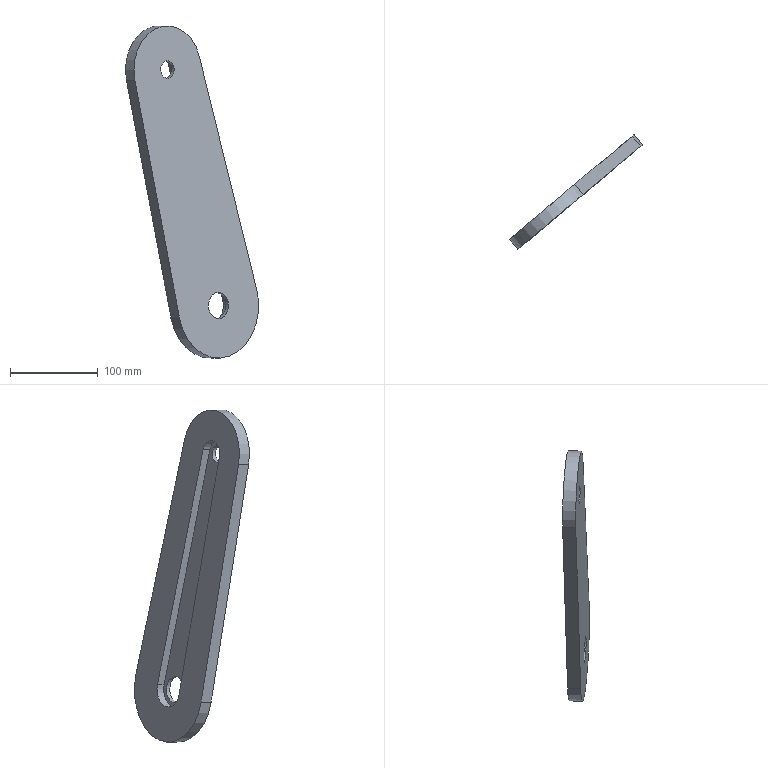Component | NX | M1002_AGO13_P09_757058_P02 | 1 solid | 13 faces | box 152.06 x 131.45 x 379.43 mm | volume 493084 mm3 | plane 7 | cylinder 6 | commonest cylinder face diameters 30 x2 20 x1 120 x1 100 x1 40 x1
STEP:
#1=CARTESIAN_POINT('',(0.,0.,0.));
#2=DIRECTION('',(0.,0.,1.));
#3=DIRECTION('',(1.,0.,0.));
#4=AXIS2_PLACEMENT_3D('',#1,#2,#3);
#5=CARTESIAN_POINT('',(13.794,-9.16,27.918));
#6=VERTEX_POINT('',#5);
#7=CARTESIAN_POINT('',(24.832,0.1404,32.));
#8=DIRECTION('',(-0.6443,0.7647,0.));
#9=DIRECTION('',(-0.7359,-0.62,-0.2721));
#10=AXIS2_PLACEMENT_3D('',#7,#8,#9);
#11=CIRCLE('',#10,15.);
#12=CARTESIAN_POINT('',(15.167,11.611,32.));
#13=DIRECTION('',(0.6443,-0.7647,0.));
#14=DIRECTION('',(-0.2081,-0.1753,0.9623));
#15=AXIS2_PLACEMENT_3D('',#12,#13,#14);
#16=CYLINDRICAL_SURFACE('',#15,15.);
#17=CARTESIAN_POINT('',(7.854,15.));
#18=DIRECTION('',(-1.,0.));
#19=VECTOR('',#18,1.);
#20=LINE('',#17,#19);
#21=(GEOMETRIC_REPRESENTATION_CONTEXT(2)PARAMETRIC_REPRESENTATION_CONTEXT()REPRESENTATION_CONTEXT('',''));
#22=DEFINITIONAL_REPRESENTATION('',(#20),#21);
#23=PCURVE('',#16,#22);
#24=CARTESIAN_POINT('',(24.832,0.1404,32.));
#25=DIRECTION('',(-0.6443,0.7647,0.));
#26=DIRECTION('',(0.2081,0.1753,-0.9623));
#27=AXIS2_PLACEMENT_3D('',#24,#25,#26);
#28=PLANE('',#27);
#29=CARTESIAN_POINT('',(0.,0.));
#30=DIRECTION('',(-0.,1.));
#31=AXIS2_PLACEMENT_2D('',#29,#30);
#32=CIRCLE('',#31,15.);
#33=(GEOMETRIC_REPRESENTATION_CONTEXT(2)PARAMETRIC_REPRESENTATION_CONTEXT()REPRESENTATION_CONTEXT('',''));
#34=DEFINITIONAL_REPRESENTATION('',(#32),#33);
#35=PCURVE('',#28,#34);
#36=SURFACE_CURVE('',#11,(#23,#35),.PCURVE_S1.);
#37=EDGE_CURVE('',#6,#6,#36,.T.);
#38=ORIENTED_EDGE('',*,*,#37,.T.);
#39=CARTESIAN_POINT('',(10.572,-5.336,27.918));
#40=VERTEX_POINT('',#39);
#41=CARTESIAN_POINT('',(10.572,-5.336,27.918));
#42=CARTESIAN_POINT('',(13.794,-9.16,27.918));
#43=B_SPLINE_CURVE_WITH_KNOTS('',1,(#41,#42),.UNSPECIFIED.,.F.,.F.,(2,2),(10.,15.),.PIECEWISE_BEZIER_KNOTS.);
#44=CARTESIAN_POINT('',(1.571,0.));
#45=DIRECTION('',(0.,1.));
#46=VECTOR('',#45,1.);
#47=LINE('',#44,#46);
#48=(GEOMETRIC_REPRESENTATION_CONTEXT(2)PARAMETRIC_REPRESENTATION_CONTEXT()REPRESENTATION_CONTEXT('',''));
#49=DEFINITIONAL_REPRESENTATION('',(#47),#48);
#50=PCURVE('',#16,#49);
#51=CARTESIAN_POINT('',(7.854,0.));
#52=DIRECTION('',(0.,1.));
#53=VECTOR('',#52,1.);
#54=LINE('',#51,#53);
#55=(GEOMETRIC_REPRESENTATION_CONTEXT(2)PARAMETRIC_REPRESENTATION_CONTEXT()REPRESENTATION_CONTEXT('',''));
#56=DEFINITIONAL_REPRESENTATION('',(#54),#55);
#57=PCURVE('',#16,#56);
#58=SEAM_CURVE('',#43,(#50,#57),.PCURVE_S1.);
#59=EDGE_CURVE('',#40,#6,#58,.T.);
#60=ORIENTED_EDGE('',*,*,#59,.F.);
#61=CARTESIAN_POINT('',(21.61,3.964,32.));
#62=DIRECTION('',(0.6443,-0.7647,-0.));
#63=DIRECTION('',(-0.7359,-0.62,-0.2721));
#64=AXIS2_PLACEMENT_3D('',#61,#62,#63);
#65=CIRCLE('',#64,15.);
#66=CARTESIAN_POINT('',(1.571,10.));
#67=DIRECTION('',(1.,0.));
#68=VECTOR('',#67,1.);
#69=LINE('',#66,#68);
#70=(GEOMETRIC_REPRESENTATION_CONTEXT(2)PARAMETRIC_REPRESENTATION_CONTEXT()REPRESENTATION_CONTEXT('',''));
#71=DEFINITIONAL_REPRESENTATION('',(#69),#70);
#72=PCURVE('',#16,#71);
#73=CARTESIAN_POINT('',(21.61,3.964,32.));
#74=DIRECTION('',(-0.6443,0.7647,0.));
#75=DIRECTION('',(0.2081,0.1753,-0.9623));
#76=AXIS2_PLACEMENT_3D('',#73,#74,#75);
#77=PLANE('',#76);
#78=CARTESIAN_POINT('',(0.,15.));
#79=CARTESIAN_POINT('',(25.981,15.));
#80=CARTESIAN_POINT('',(12.99,-7.5));
#81=CARTESIAN_POINT('',(0.,-30.));
#82=CARTESIAN_POINT('',(-12.99,-7.5));
#83=CARTESIAN_POINT('',(-25.981,15.));
#84=CARTESIAN_POINT('',(0.,15.));
#85=(BOUNDED_CURVE()B_SPLINE_CURVE(2,(#78,#79,#80,#81,#82,#83,#84),.UNSPECIFIED.,.T.,.F.)B_SPLINE_CURVE_WITH_KNOTS((1,2,2,2,2,1),(-2.094,0.,2.094,4.189,6.283,8.378),.UNSPECIFIED.)CURVE()GEOMETRIC_REPRESENTATION_ITEM()RATIONAL_B_SPLINE_CURVE((1.,0.5,1.,0.5,1.,0.5,1.))REPRESENTATION_ITEM(''));
#86=(GEOMETRIC_REPRESENTATION_CONTEXT(2)PARAMETRIC_REPRESENTATION_CONTEXT()REPRESENTATION_CONTEXT('',''));
#87=DEFINITIONAL_REPRESENTATION('',(#85),#86);
#88=PCURVE('',#77,#87);
#89=SURFACE_CURVE('',#65,(#72,#88),.PCURVE_S1.);
#90=EDGE_CURVE('',#40,#40,#89,.T.);
#91=ORIENTED_EDGE('',*,*,#90,.T.);
#92=ORIENTED_EDGE('',*,*,#59,.T.);
#93=EDGE_LOOP('',(#38,#60,#91,#92));
#94=FACE_BOUND('',#93,.F.);
#95=ADVANCED_FACE('',(#94),#16,.F.);
#96=CARTESIAN_POINT('',(-40.798,-55.157,298.711));
#97=VERTEX_POINT('',#96);
#98=CARTESIAN_POINT('',(-33.439,-48.957,301.433));
#99=DIRECTION('',(-0.6443,0.7647,0.));
#100=DIRECTION('',(-0.7359,-0.62,-0.2721));
#101=AXIS2_PLACEMENT_3D('',#98,#99,#100);
#102=CIRCLE('',#101,10.);
#103=CARTESIAN_POINT('',(-43.104,-37.486,301.433));
#104=DIRECTION('',(0.6443,-0.7647,0.));
#105=DIRECTION('',(-0.2081,-0.1753,0.9623));
#106=AXIS2_PLACEMENT_3D('',#103,#104,#105);
#107=CYLINDRICAL_SURFACE('',#106,10.);
#108=CARTESIAN_POINT('',(7.854,15.));
#109=DIRECTION('',(-1.,0.));
#110=VECTOR('',#109,1.);
#111=LINE('',#108,#110);
#112=(GEOMETRIC_REPRESENTATION_CONTEXT(2)PARAMETRIC_REPRESENTATION_CONTEXT()REPRESENTATION_CONTEXT('',''));
#113=DEFINITIONAL_REPRESENTATION('',(#111),#112);
#114=PCURVE('',#107,#113);
#115=CARTESIAN_POINT('',(-280.,0.));
#116=DIRECTION('',(-0.,1.));
#117=AXIS2_PLACEMENT_2D('',#115,#116);
#118=CIRCLE('',#117,10.);
#119=(GEOMETRIC_REPRESENTATION_CONTEXT(2)PARAMETRIC_REPRESENTATION_CONTEXT()REPRESENTATION_CONTEXT('',''));
#120=DEFINITIONAL_REPRESENTATION('',(#118),#119);
#121=PCURVE('',#28,#120);
#122=SURFACE_CURVE('',#102,(#114,#121),.PCURVE_S1.);
#123=EDGE_CURVE('',#97,#97,#122,.T.);
#124=ORIENTED_EDGE('',*,*,#123,.T.);
#125=CARTESIAN_POINT('',(-44.019,-51.333,298.711));
#126=VERTEX_POINT('',#125);
#127=CARTESIAN_POINT('',(-44.019,-51.333,298.711));
#128=CARTESIAN_POINT('',(-40.798,-55.157,298.711));
#129=B_SPLINE_CURVE_WITH_KNOTS('',1,(#127,#128),.UNSPECIFIED.,.F.,.F.,(2,2),(10.,15.),.PIECEWISE_BEZIER_KNOTS.);
#130=CARTESIAN_POINT('',(1.571,0.));
#131=DIRECTION('',(0.,1.));
#132=VECTOR('',#131,1.);
#133=LINE('',#130,#132);
#134=(GEOMETRIC_REPRESENTATION_CONTEXT(2)PARAMETRIC_REPRESENTATION_CONTEXT()REPRESENTATION_CONTEXT('',''));
#135=DEFINITIONAL_REPRESENTATION('',(#133),#134);
#136=PCURVE('',#107,#135);
#137=CARTESIAN_POINT('',(7.854,0.));
#138=DIRECTION('',(0.,1.));
#139=VECTOR('',#138,1.);
#140=LINE('',#137,#139);
#141=(GEOMETRIC_REPRESENTATION_CONTEXT(2)PARAMETRIC_REPRESENTATION_CONTEXT()REPRESENTATION_CONTEXT('',''));
#142=DEFINITIONAL_REPRESENTATION('',(#140),#141);
#143=PCURVE('',#107,#142);
#144=SEAM_CURVE('',#129,(#136,#143),.PCURVE_S1.);
#145=EDGE_CURVE('',#126,#97,#144,.T.);
#146=ORIENTED_EDGE('',*,*,#145,.F.);
#147=CARTESIAN_POINT('',(-36.661,-45.133,301.433));
#148=DIRECTION('',(0.6443,-0.7647,-0.));
#149=DIRECTION('',(-0.7359,-0.62,-0.2721));
#150=AXIS2_PLACEMENT_3D('',#147,#148,#149);
#151=CIRCLE('',#150,10.);
#152=CARTESIAN_POINT('',(1.571,10.));
#153=DIRECTION('',(1.,0.));
#154=VECTOR('',#153,1.);
#155=LINE('',#152,#154);
#156=(GEOMETRIC_REPRESENTATION_CONTEXT(2)PARAMETRIC_REPRESENTATION_CONTEXT()REPRESENTATION_CONTEXT('',''));
#157=DEFINITIONAL_REPRESENTATION('',(#155),#156);
#158=PCURVE('',#107,#157);
#159=CARTESIAN_POINT('',(-280.,10.));
#160=CARTESIAN_POINT('',(-262.679,10.));
#161=CARTESIAN_POINT('',(-271.34,-5.));
#162=CARTESIAN_POINT('',(-280.,-20.));
#163=CARTESIAN_POINT('',(-288.66,-5.));
#164=CARTESIAN_POINT('',(-297.321,10.));
#165=CARTESIAN_POINT('',(-280.,10.));
#166=(BOUNDED_CURVE()B_SPLINE_CURVE(2,(#159,#160,#161,#162,#163,#164,#165),.UNSPECIFIED.,.T.,.F.)B_SPLINE_CURVE_WITH_KNOTS((1,2,2,2,2,1),(-2.094,0.,2.094,4.189,6.283,8.378),.UNSPECIFIED.)CURVE()GEOMETRIC_REPRESENTATION_ITEM()RATIONAL_B_SPLINE_CURVE((1.,0.5,1.,0.5,1.,0.5,1.))REPRESENTATION_ITEM(''));
#167=(GEOMETRIC_REPRESENTATION_CONTEXT(2)PARAMETRIC_REPRESENTATION_CONTEXT()REPRESENTATION_CONTEXT('',''));
#168=DEFINITIONAL_REPRESENTATION('',(#166),#167);
#169=PCURVE('',#77,#168);
#170=SURFACE_CURVE('',#151,(#158,#169),.PCURVE_S1.);
#171=EDGE_CURVE('',#126,#126,#170,.T.);
#172=ORIENTED_EDGE('',*,*,#171,.T.);
#173=ORIENTED_EDGE('',*,*,#145,.T.);
#174=EDGE_LOOP('',(#124,#146,#172,#173));
#175=FACE_BOUND('',#174,.F.);
#176=ADVANCED_FACE('',(#175),#107,.F.);
#177=CARTESIAN_POINT('',(68.51,36.942,50.38));
#178=VERTEX_POINT('',#177);
#179=CARTESIAN_POINT('',(-19.739,-37.413,17.744));
#180=VERTEX_POINT('',#179);
#181=CARTESIAN_POINT('',(24.832,0.1404,32.));
#182=DIRECTION('',(-0.6443,0.7647,0.));
#183=DIRECTION('',(-0.7359,-0.62,-0.2721));
#184=AXIS2_PLACEMENT_3D('',#181,#182,#183);
#185=CIRCLE('',#184,60.);
#186=CARTESIAN_POINT('',(15.167,11.611,32.));
#187=DIRECTION('',(0.6443,-0.7647,0.));
#188=DIRECTION('',(-0.2081,-0.1753,0.9623));
#189=AXIS2_PLACEMENT_3D('',#186,#187,#188);
#190=CYLINDRICAL_SURFACE('',#189,60.);
#191=CARTESIAN_POINT('',(7.854,15.));
#192=DIRECTION('',(-1.,-0.));
#193=VECTOR('',#192,1.);
#194=LINE('',#191,#193);
#195=(GEOMETRIC_REPRESENTATION_CONTEXT(2)PARAMETRIC_REPRESENTATION_CONTEXT()REPRESENTATION_CONTEXT('',''));
#196=DEFINITIONAL_REPRESENTATION('',(#194),#195);
#197=PCURVE('',#190,#196);
#198=CARTESIAN_POINT('',(0.,0.));
#199=DIRECTION('',(-0.,1.));
#200=AXIS2_PLACEMENT_2D('',#198,#199);
#201=CIRCLE('',#200,60.);
#202=(GEOMETRIC_REPRESENTATION_CONTEXT(2)PARAMETRIC_REPRESENTATION_CONTEXT()REPRESENTATION_CONTEXT('',''));
#203=DEFINITIONAL_REPRESENTATION('',(#201),#202);
#204=PCURVE('',#28,#203);
#205=SURFACE_CURVE('',#185,(#197,#204),.PCURVE_S1.);
#206=EDGE_CURVE('',#178,#180,#205,.T.);
#207=ORIENTED_EDGE('',*,*,#206,.T.);
#208=CARTESIAN_POINT('',(-29.404,-25.942,17.744));
#209=VERTEX_POINT('',#208);
#210=CARTESIAN_POINT('',(-29.404,-25.942,17.744));
#211=DIRECTION('',(0.6443,-0.7647,0.));
#212=VECTOR('',#211,1.);
#213=LINE('',#210,#212);
#214=CARTESIAN_POINT('',(1.535,-0.));
#215=DIRECTION('',(0.,1.));
#216=VECTOR('',#215,1.);
#217=LINE('',#214,#216);
#218=(GEOMETRIC_REPRESENTATION_CONTEXT(2)PARAMETRIC_REPRESENTATION_CONTEXT()REPRESENTATION_CONTEXT('',''));
#219=DEFINITIONAL_REPRESENTATION('',(#217),#218);
#220=PCURVE('',#190,#219);
#221=CARTESIAN_POINT('',(-29.404,-25.942,17.744));
#222=DIRECTION('',(0.7428,0.6259,0.2376));
#223=DIRECTION('',(0.1817,0.1531,-0.9714));
#224=AXIS2_PLACEMENT_3D('',#221,#222,#223);
#225=PLANE('',#224);
#226=CARTESIAN_POINT('',(-0.,-0.));
#227=DIRECTION('',(0.,-1.));
#228=VECTOR('',#227,1.);
#229=LINE('',#226,#228);
#230=(GEOMETRIC_REPRESENTATION_CONTEXT(2)PARAMETRIC_REPRESENTATION_CONTEXT()REPRESENTATION_CONTEXT('',''));
#231=DEFINITIONAL_REPRESENTATION('',(#229),#230);
#232=PCURVE('',#225,#231);
#233=SURFACE_CURVE('',#213,(#220,#232),.PCURVE_S1.);
#234=EDGE_CURVE('',#209,#180,#233,.T.);
#235=ORIENTED_EDGE('',*,*,#234,.F.);
#236=CARTESIAN_POINT('',(58.845,48.413,50.38));
#237=VERTEX_POINT('',#236);
#238=CARTESIAN_POINT('',(15.167,11.611,32.));
#239=DIRECTION('',(-0.6443,0.7647,0.));
#240=DIRECTION('',(-0.7359,-0.62,-0.2721));
#241=AXIS2_PLACEMENT_3D('',#238,#239,#240);
#242=CIRCLE('',#241,60.);
#243=CARTESIAN_POINT('',(7.854,0.));
#244=DIRECTION('',(-1.,-0.));
#245=VECTOR('',#244,1.);
#246=LINE('',#243,#245);
#247=(GEOMETRIC_REPRESENTATION_CONTEXT(2)PARAMETRIC_REPRESENTATION_CONTEXT()REPRESENTATION_CONTEXT('',''));
#248=DEFINITIONAL_REPRESENTATION('',(#246),#247);
#249=PCURVE('',#190,#248);
#250=CARTESIAN_POINT('',(15.167,11.611,32.));
#251=DIRECTION('',(-0.6443,0.7647,0.));
#252=DIRECTION('',(0.2081,0.1753,-0.9623));
#253=AXIS2_PLACEMENT_3D('',#250,#251,#252);
#254=PLANE('',#253);
#255=CARTESIAN_POINT('',(0.,0.));
#256=DIRECTION('',(-0.,1.));
#257=AXIS2_PLACEMENT_2D('',#255,#256);
#258=CIRCLE('',#257,60.);
#259=(GEOMETRIC_REPRESENTATION_CONTEXT(2)PARAMETRIC_REPRESENTATION_CONTEXT()REPRESENTATION_CONTEXT('',''));
#260=DEFINITIONAL_REPRESENTATION('',(#258),#259);
#261=PCURVE('',#254,#260);
#262=SURFACE_CURVE('',#242,(#249,#261),.PCURVE_S1.);
#263=EDGE_CURVE('',#237,#209,#262,.T.);
#264=ORIENTED_EDGE('',*,*,#263,.F.);
#265=CARTESIAN_POINT('',(58.845,48.413,50.38));
#266=DIRECTION('',(0.6443,-0.7647,0.));
#267=VECTOR('',#266,1.);
#268=LINE('',#265,#267);
#269=CARTESIAN_POINT('',(4.748,0.));
#270=DIRECTION('',(0.,1.));
#271=VECTOR('',#270,1.);
#272=LINE('',#269,#271);
#273=(GEOMETRIC_REPRESENTATION_CONTEXT(2)PARAMETRIC_REPRESENTATION_CONTEXT()REPRESENTATION_CONTEXT('',''));
#274=DEFINITIONAL_REPRESENTATION('',(#272),#273);
#275=PCURVE('',#190,#274);
#276=CARTESIAN_POINT('',(-6.705,-6.817,316.749));
#277=DIRECTION('',(-0.728,-0.6134,-0.3063));
#278=DIRECTION('',(-0.2343,-0.1974,0.9519));
#279=AXIS2_PLACEMENT_3D('',#276,#277,#278);
#280=PLANE('',#279);
#281=CARTESIAN_POINT('',(-279.821,0.));
#282=DIRECTION('',(-0.,-1.));
#283=VECTOR('',#282,1.);
#284=LINE('',#281,#283);
#285=(GEOMETRIC_REPRESENTATION_CONTEXT(2)PARAMETRIC_REPRESENTATION_CONTEXT()REPRESENTATION_CONTEXT('',''));
#286=DEFINITIONAL_REPRESENTATION('',(#284),#285);
#287=PCURVE('',#280,#286);
#288=SURFACE_CURVE('',#268,(#275,#287),.PCURVE_S1.);
#289=EDGE_CURVE('',#237,#178,#288,.T.);
#290=ORIENTED_EDGE('',*,*,#289,.T.);
#291=EDGE_LOOP('',(#207,#235,#264,#290));
#292=FACE_BOUND('',#291,.T.);
#293=ADVANCED_FACE('',(#292),#190,.T.);
#294=CARTESIAN_POINT('',(-70.581,-80.251,289.553));
#295=VERTEX_POINT('',#294);
#296=CARTESIAN_POINT('',(-19.739,-37.413,17.744));
#297=DIRECTION('',(-0.1817,-0.1531,0.9714));
#298=VECTOR('',#297,1.);
#299=LINE('',#296,#298);
#300=CARTESIAN_POINT('',(0.,-15.));
#301=DIRECTION('',(-1.,0.));
#302=VECTOR('',#301,1.);
#303=LINE('',#300,#302);
#304=(GEOMETRIC_REPRESENTATION_CONTEXT(2)PARAMETRIC_REPRESENTATION_CONTEXT()REPRESENTATION_CONTEXT('',''));
#305=DEFINITIONAL_REPRESENTATION('',(#303),#304);
#306=PCURVE('',#225,#305);
#307=CARTESIAN_POINT('',(-2.143,59.962));
#308=DIRECTION('',(-0.9994,-0.03571));
#309=VECTOR('',#308,1.);
#310=LINE('',#307,#309);
#311=(GEOMETRIC_REPRESENTATION_CONTEXT(2)PARAMETRIC_REPRESENTATION_CONTEXT()REPRESENTATION_CONTEXT('',''));
#312=DEFINITIONAL_REPRESENTATION('',(#310),#311);
#313=PCURVE('',#28,#312);
#314=SURFACE_CURVE('',#299,(#306,#313),.PCURVE_S1.);
#315=EDGE_CURVE('',#180,#295,#314,.T.);
#316=ORIENTED_EDGE('',*,*,#315,.T.);
#317=CARTESIAN_POINT('',(-80.246,-68.78,289.553));
#318=VERTEX_POINT('',#317);
#319=CARTESIAN_POINT('',(-80.246,-68.78,289.553));
#320=DIRECTION('',(0.6443,-0.7647,0.));
#321=VECTOR('',#320,1.);
#322=LINE('',#319,#321);
#323=CARTESIAN_POINT('',(-279.821,-0.));
#324=DIRECTION('',(0.,-1.));
#325=VECTOR('',#324,1.);
#326=LINE('',#323,#325);
#327=(GEOMETRIC_REPRESENTATION_CONTEXT(2)PARAMETRIC_REPRESENTATION_CONTEXT()REPRESENTATION_CONTEXT('',''));
#328=DEFINITIONAL_REPRESENTATION('',(#326),#327);
#329=PCURVE('',#225,#328);
#330=CARTESIAN_POINT('',(-43.104,-37.486,301.433));
#331=DIRECTION('',(0.6443,-0.7647,0.));
#332=DIRECTION('',(-0.2081,-0.1753,0.9623));
#333=AXIS2_PLACEMENT_3D('',#330,#331,#332);
#334=CYLINDRICAL_SURFACE('',#333,50.);
#335=CARTESIAN_POINT('',(1.535,0.));
#336=DIRECTION('',(0.,1.));
#337=VECTOR('',#336,1.);
#338=LINE('',#335,#337);
#339=(GEOMETRIC_REPRESENTATION_CONTEXT(2)PARAMETRIC_REPRESENTATION_CONTEXT()REPRESENTATION_CONTEXT('',''));
#340=DEFINITIONAL_REPRESENTATION('',(#338),#339);
#341=PCURVE('',#334,#340);
#342=SURFACE_CURVE('',#322,(#329,#341),.PCURVE_S1.);
#343=EDGE_CURVE('',#318,#295,#342,.T.);
#344=ORIENTED_EDGE('',*,*,#343,.F.);
#345=CARTESIAN_POINT('',(-29.404,-25.942,17.744));
#346=DIRECTION('',(-0.1817,-0.1531,0.9714));
#347=VECTOR('',#346,1.);
#348=LINE('',#345,#347);
#349=CARTESIAN_POINT('',(0.,0.));
#350=DIRECTION('',(-1.,0.));
#351=VECTOR('',#350,1.);
#352=LINE('',#349,#351);
#353=(GEOMETRIC_REPRESENTATION_CONTEXT(2)PARAMETRIC_REPRESENTATION_CONTEXT()REPRESENTATION_CONTEXT('',''));
#354=DEFINITIONAL_REPRESENTATION('',(#352),#353);
#355=PCURVE('',#225,#354);
#356=CARTESIAN_POINT('',(-2.143,59.962));
#357=DIRECTION('',(-0.9994,-0.03571));
#358=VECTOR('',#357,1.);
#359=LINE('',#356,#358);
#360=(GEOMETRIC_REPRESENTATION_CONTEXT(2)PARAMETRIC_REPRESENTATION_CONTEXT()REPRESENTATION_CONTEXT('',''));
#361=DEFINITIONAL_REPRESENTATION('',(#359),#360);
#362=PCURVE('',#254,#361);
#363=SURFACE_CURVE('',#348,(#355,#362),.PCURVE_S1.);
#364=EDGE_CURVE('',#209,#318,#363,.T.);
#365=ORIENTED_EDGE('',*,*,#364,.F.);
#366=ORIENTED_EDGE('',*,*,#234,.T.);
#367=EDGE_LOOP('',(#316,#344,#365,#366));
#368=FACE_BOUND('',#367,.T.);
#369=ADVANCED_FACE('',(#368),#225,.F.);
#370=CARTESIAN_POINT('',(2.96,-18.288,316.749));
#371=VERTEX_POINT('',#370);
#372=CARTESIAN_POINT('',(-33.439,-48.957,301.433));
#373=DIRECTION('',(-0.6443,0.7647,0.));
#374=DIRECTION('',(-0.7359,-0.62,-0.2721));
#375=AXIS2_PLACEMENT_3D('',#372,#373,#374);
#376=CIRCLE('',#375,50.);
#377=CARTESIAN_POINT('',(1.571,15.));
#378=DIRECTION('',(-1.,0.));
#379=VECTOR('',#378,1.);
#380=LINE('',#377,#379);
#381=(GEOMETRIC_REPRESENTATION_CONTEXT(2)PARAMETRIC_REPRESENTATION_CONTEXT()REPRESENTATION_CONTEXT('',''));
#382=DEFINITIONAL_REPRESENTATION('',(#380),#381);
#383=PCURVE('',#334,#382);
#384=CARTESIAN_POINT('',(-280.,0.));
#385=DIRECTION('',(-0.,1.));
#386=AXIS2_PLACEMENT_2D('',#384,#385);
#387=CIRCLE('',#386,50.);
#388=(GEOMETRIC_REPRESENTATION_CONTEXT(2)PARAMETRIC_REPRESENTATION_CONTEXT()REPRESENTATION_CONTEXT('',''));
#389=DEFINITIONAL_REPRESENTATION('',(#387),#388);
#390=PCURVE('',#28,#389);
#391=SURFACE_CURVE('',#376,(#383,#390),.PCURVE_S1.);
#392=EDGE_CURVE('',#295,#371,#391,.T.);
#393=ORIENTED_EDGE('',*,*,#392,.T.);
#394=CARTESIAN_POINT('',(-6.705,-6.817,316.749));
#395=VERTEX_POINT('',#394);
#396=CARTESIAN_POINT('',(-6.705,-6.817,316.749));
#397=DIRECTION('',(0.6443,-0.7647,0.));
#398=VECTOR('',#397,1.);
#399=LINE('',#396,#398);
#400=CARTESIAN_POINT('',(-1.535,0.));
#401=DIRECTION('',(0.,1.));
#402=VECTOR('',#401,1.);
#403=LINE('',#400,#402);
#404=(GEOMETRIC_REPRESENTATION_CONTEXT(2)PARAMETRIC_REPRESENTATION_CONTEXT()REPRESENTATION_CONTEXT('',''));
#405=DEFINITIONAL_REPRESENTATION('',(#403),#404);
#406=PCURVE('',#334,#405);
#407=CARTESIAN_POINT('',(0.,-0.));
#408=DIRECTION('',(-0.,-1.));
#409=VECTOR('',#408,1.);
#410=LINE('',#407,#409);
#411=(GEOMETRIC_REPRESENTATION_CONTEXT(2)PARAMETRIC_REPRESENTATION_CONTEXT()REPRESENTATION_CONTEXT('',''));
#412=DEFINITIONAL_REPRESENTATION('',(#410),#411);
#413=PCURVE('',#280,#412);
#414=SURFACE_CURVE('',#399,(#406,#413),.PCURVE_S1.);
#415=EDGE_CURVE('',#395,#371,#414,.T.);
#416=ORIENTED_EDGE('',*,*,#415,.F.);
#417=CARTESIAN_POINT('',(-43.104,-37.486,301.433));
#418=DIRECTION('',(-0.6443,0.7647,0.));
#419=DIRECTION('',(-0.7359,-0.62,-0.2721));
#420=AXIS2_PLACEMENT_3D('',#417,#418,#419);
#421=CIRCLE('',#420,50.);
#422=CARTESIAN_POINT('',(1.571,0.));
#423=DIRECTION('',(-1.,-0.));
#424=VECTOR('',#423,1.);
#425=LINE('',#422,#424);
#426=(GEOMETRIC_REPRESENTATION_CONTEXT(2)PARAMETRIC_REPRESENTATION_CONTEXT()REPRESENTATION_CONTEXT('',''));
#427=DEFINITIONAL_REPRESENTATION('',(#425),#426);
#428=PCURVE('',#334,#427);
#429=CARTESIAN_POINT('',(-280.,-0.));
#430=DIRECTION('',(-0.,1.));
#431=AXIS2_PLACEMENT_2D('',#429,#430);
#432=CIRCLE('',#431,50.);
#433=(GEOMETRIC_REPRESENTATION_CONTEXT(2)PARAMETRIC_REPRESENTATION_CONTEXT()REPRESENTATION_CONTEXT('',''));
#434=DEFINITIONAL_REPRESENTATION('',(#432),#433);
#435=PCURVE('',#254,#434);
#436=SURFACE_CURVE('',#421,(#428,#435),.PCURVE_S1.);
#437=EDGE_CURVE('',#318,#395,#436,.T.);
#438=ORIENTED_EDGE('',*,*,#437,.F.);
#439=ORIENTED_EDGE('',*,*,#343,.T.);
#440=EDGE_LOOP('',(#393,#416,#438,#439));
#441=FACE_BOUND('',#440,.T.);
#442=ADVANCED_FACE('',(#441),#334,.T.);
#443=CARTESIAN_POINT('',(2.96,-18.288,316.749));
#444=DIRECTION('',(0.2343,0.1974,-0.9519));
#445=VECTOR('',#444,1.);
#446=LINE('',#443,#445);
#447=CARTESIAN_POINT('',(-0.,-15.));
#448=DIRECTION('',(-1.,-0.));
#449=VECTOR('',#448,1.);
#450=LINE('',#447,#449);
#451=(GEOMETRIC_REPRESENTATION_CONTEXT(2)PARAMETRIC_REPRESENTATION_CONTEXT()REPRESENTATION_CONTEXT('',''));
#452=DEFINITIONAL_REPRESENTATION('',(#450),#451);
#453=PCURVE('',#280,#452);
#454=CARTESIAN_POINT('',(-281.786,-49.968));
#455=DIRECTION('',(0.9994,-0.03571));
#456=VECTOR('',#455,1.);
#457=LINE('',#454,#456);
#458=(GEOMETRIC_REPRESENTATION_CONTEXT(2)PARAMETRIC_REPRESENTATION_CONTEXT()REPRESENTATION_CONTEXT('',''));
#459=DEFINITIONAL_REPRESENTATION('',(#457),#458);
#460=PCURVE('',#28,#459);
#461=SURFACE_CURVE('',#446,(#453,#460),.PCURVE_S1.);
#462=EDGE_CURVE('',#371,#178,#461,.T.);
#463=ORIENTED_EDGE('',*,*,#462,.T.);
#464=ORIENTED_EDGE('',*,*,#289,.F.);
#465=CARTESIAN_POINT('',(-6.705,-6.817,316.749));
#466=DIRECTION('',(0.2343,0.1974,-0.9519));
#467=VECTOR('',#466,1.);
#468=LINE('',#465,#467);
#469=CARTESIAN_POINT('',(0.,0.));
#470=DIRECTION('',(-1.,-0.));
#471=VECTOR('',#470,1.);
#472=LINE('',#469,#471);
#473=(GEOMETRIC_REPRESENTATION_CONTEXT(2)PARAMETRIC_REPRESENTATION_CONTEXT()REPRESENTATION_CONTEXT('',''));
#474=DEFINITIONAL_REPRESENTATION('',(#472),#473);
#475=PCURVE('',#280,#474);
#476=CARTESIAN_POINT('',(-281.786,-49.968));
#477=DIRECTION('',(0.9994,-0.03571));
#478=VECTOR('',#477,1.);
#479=LINE('',#476,#478);
#480=(GEOMETRIC_REPRESENTATION_CONTEXT(2)PARAMETRIC_REPRESENTATION_CONTEXT()REPRESENTATION_CONTEXT('',''));
#481=DEFINITIONAL_REPRESENTATION('',(#479),#480);
#482=PCURVE('',#254,#481);
#483=SURFACE_CURVE('',#468,(#475,#482),.PCURVE_S1.);
#484=EDGE_CURVE('',#395,#237,#483,.T.);
#485=ORIENTED_EDGE('',*,*,#484,.F.);
#486=ORIENTED_EDGE('',*,*,#415,.T.);
#487=EDGE_LOOP('',(#463,#464,#485,#486));
#488=FACE_BOUND('',#487,.T.);
#489=ADVANCED_FACE('',(#488),#280,.F.);
#490=CARTESIAN_POINT('',(29.807,23.947,37.785));
#491=VERTEX_POINT('',#490);
#492=CARTESIAN_POINT('',(0.3771,-0.8497,26.902));
#493=VERTEX_POINT('',#492);
#494=CARTESIAN_POINT('',(15.167,11.611,32.));
#495=DIRECTION('',(-0.6443,0.7647,0.));
#496=DIRECTION('',(-0.7428,-0.6259,-0.2376));
#497=AXIS2_PLACEMENT_3D('',#494,#495,#496);
#498=CIRCLE('',#497,20.);
#499=CARTESIAN_POINT('',(-0.,-0.));
#500=DIRECTION('',(-0.03571,0.9994));
#501=AXIS2_PLACEMENT_2D('',#499,#500);
#502=CIRCLE('',#501,20.);
#503=(GEOMETRIC_REPRESENTATION_CONTEXT(2)PARAMETRIC_REPRESENTATION_CONTEXT()REPRESENTATION_CONTEXT('',''));
#504=DEFINITIONAL_REPRESENTATION('',(#502),#503);
#505=PCURVE('',#254,#504);
#506=CARTESIAN_POINT('',(21.61,3.964,32.));
#507=DIRECTION('',(-0.6443,0.7647,0.));
#508=DIRECTION('',(0.2081,0.1753,-0.9623));
#509=AXIS2_PLACEMENT_3D('',#506,#507,#508);
#510=CYLINDRICAL_SURFACE('',#509,20.);
#511=CARTESIAN_POINT('',(1.607,10.));
#512=DIRECTION('',(1.,0.));
#513=VECTOR('',#512,1.);
#514=LINE('',#511,#513);
#515=(GEOMETRIC_REPRESENTATION_CONTEXT(2)PARAMETRIC_REPRESENTATION_CONTEXT()REPRESENTATION_CONTEXT('',''));
#516=DEFINITIONAL_REPRESENTATION('',(#514),#515);
#517=PCURVE('',#510,#516);
#518=SURFACE_CURVE('',#498,(#505,#517),.PCURVE_S1.);
#519=EDGE_CURVE('',#491,#493,#518,.T.);
#520=ORIENTED_EDGE('',*,*,#519,.F.);
#521=CARTESIAN_POINT('',(-32.123,-28.234,305.772));
#522=VERTEX_POINT('',#521);
#523=CARTESIAN_POINT('',(-32.123,-28.234,305.772));
#524=DIRECTION('',(0.2212,0.1864,-0.9572));
#525=VECTOR('',#524,1.);
#526=LINE('',#523,#525);
#527=CARTESIAN_POINT('',(-280.268,-14.998));
#528=DIRECTION('',(0.9998,-0.01786));
#529=VECTOR('',#528,1.);
#530=LINE('',#527,#529);
#531=(GEOMETRIC_REPRESENTATION_CONTEXT(2)PARAMETRIC_REPRESENTATION_CONTEXT()REPRESENTATION_CONTEXT('',''));
#532=DEFINITIONAL_REPRESENTATION('',(#530),#531);
#533=PCURVE('',#254,#532);
#534=CARTESIAN_POINT('',(-25.68,-35.881,305.772));
#535=DIRECTION('',(0.732,0.6168,0.2893));
#536=DIRECTION('',(0.2212,0.1864,-0.9572));
#537=AXIS2_PLACEMENT_3D('',#534,#535,#536);
#538=PLANE('',#537);
#539=CARTESIAN_POINT('',(-0.,10.));
#540=DIRECTION('',(1.,0.));
#541=VECTOR('',#540,1.);
#542=LINE('',#539,#541);
#543=(GEOMETRIC_REPRESENTATION_CONTEXT(2)PARAMETRIC_REPRESENTATION_CONTEXT()REPRESENTATION_CONTEXT('',''));
#544=DEFINITIONAL_REPRESENTATION('',(#542),#543);
#545=PCURVE('',#538,#544);
#546=SURFACE_CURVE('',#526,(#533,#545),.PCURVE_S1.);
#547=EDGE_CURVE('',#522,#491,#546,.T.);
#548=ORIENTED_EDGE('',*,*,#547,.F.);
#549=CARTESIAN_POINT('',(-54.196,-46.831,297.609));
#550=VERTEX_POINT('',#549);
#551=CARTESIAN_POINT('',(-43.104,-37.486,301.433));
#552=DIRECTION('',(-0.6443,0.7647,0.));
#553=DIRECTION('',(-0.7428,-0.6259,-0.2376));
#554=AXIS2_PLACEMENT_3D('',#551,#552,#553);
#555=CIRCLE('',#554,15.);
#556=CARTESIAN_POINT('',(-280.,-0.));
#557=DIRECTION('',(-0.03571,0.9994));
#558=AXIS2_PLACEMENT_2D('',#556,#557);
#559=CIRCLE('',#558,15.);
#560=(GEOMETRIC_REPRESENTATION_CONTEXT(2)PARAMETRIC_REPRESENTATION_CONTEXT()REPRESENTATION_CONTEXT('',''));
#561=DEFINITIONAL_REPRESENTATION('',(#559),#560);
#562=PCURVE('',#254,#561);
#563=CARTESIAN_POINT('',(-36.661,-45.133,301.433));
#564=DIRECTION('',(-0.6443,0.7647,0.));
#565=DIRECTION('',(0.2081,0.1753,-0.9623));
#566=AXIS2_PLACEMENT_3D('',#563,#564,#565);
#567=CYLINDRICAL_SURFACE('',#566,15.);
#568=CARTESIAN_POINT('',(-4.677,10.));
#569=DIRECTION('',(1.,-0.));
#570=VECTOR('',#569,1.);
#571=LINE('',#568,#570);
#572=(GEOMETRIC_REPRESENTATION_CONTEXT(2)PARAMETRIC_REPRESENTATION_CONTEXT()REPRESENTATION_CONTEXT('',''));
#573=DEFINITIONAL_REPRESENTATION('',(#571),#572);
#574=PCURVE('',#567,#573);
#575=SURFACE_CURVE('',#555,(#562,#574),.PCURVE_S1.);
#576=EDGE_CURVE('',#550,#522,#575,.T.);
#577=ORIENTED_EDGE('',*,*,#576,.F.);
#578=CARTESIAN_POINT('',(0.3771,-0.8497,26.902));
#579=DIRECTION('',(-0.1949,-0.1642,0.967));
#580=VECTOR('',#579,1.);
#581=LINE('',#578,#580);
#582=CARTESIAN_POINT('',(-0.3571,19.997));
#583=DIRECTION('',(-0.9998,-0.01786));
#584=VECTOR('',#583,1.);
#585=LINE('',#582,#584);
#586=(GEOMETRIC_REPRESENTATION_CONTEXT(2)PARAMETRIC_REPRESENTATION_CONTEXT()REPRESENTATION_CONTEXT('',''));
#587=DEFINITIONAL_REPRESENTATION('',(#585),#586);
#588=PCURVE('',#254,#587);
#589=CARTESIAN_POINT('',(6.821,-8.497,26.902));
#590=DIRECTION('',(-0.7395,-0.6231,-0.2549));
#591=DIRECTION('',(-0.1949,-0.1642,0.967));
#592=AXIS2_PLACEMENT_3D('',#589,#590,#591);
#593=PLANE('',#592);
#594=CARTESIAN_POINT('',(0.,10.));
#595=DIRECTION('',(1.,0.));
#596=VECTOR('',#595,1.);
#597=LINE('',#594,#596);
#598=(GEOMETRIC_REPRESENTATION_CONTEXT(2)PARAMETRIC_REPRESENTATION_CONTEXT()REPRESENTATION_CONTEXT('',''));
#599=DEFINITIONAL_REPRESENTATION('',(#597),#598);
#600=PCURVE('',#593,#599);
#601=SURFACE_CURVE('',#581,(#588,#600),.PCURVE_S1.);
#602=EDGE_CURVE('',#493,#550,#601,.T.);
#603=ORIENTED_EDGE('',*,*,#602,.F.);
#604=EDGE_LOOP('',(#520,#548,#577,#603));
#605=FACE_BOUND('',#604,.T.);
#606=ORIENTED_EDGE('',*,*,#263,.T.);
#607=ORIENTED_EDGE('',*,*,#364,.T.);
#608=ORIENTED_EDGE('',*,*,#437,.T.);
#609=ORIENTED_EDGE('',*,*,#484,.T.);
#610=EDGE_LOOP('',(#606,#607,#608,#609));
#611=FACE_BOUND('',#610,.T.);
#612=ADVANCED_FACE('',(#605,#611),#254,.T.);
#613=ORIENTED_EDGE('',*,*,#206,.F.);
#614=ORIENTED_EDGE('',*,*,#462,.F.);
#615=ORIENTED_EDGE('',*,*,#392,.F.);
#616=ORIENTED_EDGE('',*,*,#315,.F.);
#617=EDGE_LOOP('',(#613,#614,#615,#616));
#618=FACE_BOUND('',#617,.T.);
#619=ORIENTED_EDGE('',*,*,#37,.T.);
#620=EDGE_LOOP('',(#619));
#621=FACE_BOUND('',#620,.T.);
#622=ORIENTED_EDGE('',*,*,#123,.T.);
#623=EDGE_LOOP('',(#622));
#624=FACE_BOUND('',#623,.T.);
#625=ADVANCED_FACE('',(#618,#621,#624),#28,.F.);
#626=CARTESIAN_POINT('',(36.251,16.3,37.785));
#627=VERTEX_POINT('',#626);
#628=CARTESIAN_POINT('',(36.251,16.3,37.785));
#629=DIRECTION('',(0.6443,-0.7647,0.));
#630=VECTOR('',#629,1.);
#631=LINE('',#628,#630);
#632=CARTESIAN_POINT('',(4.695,0.));
#633=DIRECTION('',(0.,-1.));
#634=VECTOR('',#633,1.);
#635=LINE('',#632,#634);
#636=(GEOMETRIC_REPRESENTATION_CONTEXT(2)PARAMETRIC_REPRESENTATION_CONTEXT()REPRESENTATION_CONTEXT('',''));
#637=DEFINITIONAL_REPRESENTATION('',(#635),#636);
#638=PCURVE('',#510,#637);
#639=CARTESIAN_POINT('',(279.955,-0.));
#640=DIRECTION('',(0.,-1.));
#641=VECTOR('',#640,1.);
#642=LINE('',#639,#641);
#643=(GEOMETRIC_REPRESENTATION_CONTEXT(2)PARAMETRIC_REPRESENTATION_CONTEXT()REPRESENTATION_CONTEXT('',''));
#644=DEFINITIONAL_REPRESENTATION('',(#642),#643);
#645=PCURVE('',#538,#644);
#646=SURFACE_CURVE('',#631,(#638,#645),.PCURVE_S1.);
#647=EDGE_CURVE('',#491,#627,#646,.T.);
#648=ORIENTED_EDGE('',*,*,#647,.T.);
#649=CARTESIAN_POINT('',(6.821,-8.497,26.902));
#650=VERTEX_POINT('',#649);
#651=CARTESIAN_POINT('',(21.61,3.964,32.));
#652=DIRECTION('',(0.6443,-0.7647,-0.));
#653=DIRECTION('',(-0.7428,-0.6259,-0.2376));
#654=AXIS2_PLACEMENT_3D('',#651,#652,#653);
#655=CIRCLE('',#654,20.);
#656=CARTESIAN_POINT('',(7.89,-0.));
#657=DIRECTION('',(-1.,0.));
#658=VECTOR('',#657,1.);
#659=LINE('',#656,#658);
#660=(GEOMETRIC_REPRESENTATION_CONTEXT(2)PARAMETRIC_REPRESENTATION_CONTEXT()REPRESENTATION_CONTEXT('',''));
#661=DEFINITIONAL_REPRESENTATION('',(#659),#660);
#662=PCURVE('',#510,#661);
#663=CARTESIAN_POINT('',(-0.7143,19.987));
#664=CARTESIAN_POINT('',(33.905,21.224));
#665=CARTESIAN_POINT('',(17.667,-9.375));
#666=CARTESIAN_POINT('',(1.429,-39.974));
#667=CARTESIAN_POINT('',(-16.952,-10.612));
#668=CARTESIAN_POINT('',(-35.333,18.75));
#669=CARTESIAN_POINT('',(-0.7143,19.987));
#670=(BOUNDED_CURVE()B_SPLINE_CURVE(2,(#663,#664,#665,#666,#667,#668,#669),.UNSPECIFIED.,.T.,.F.)B_SPLINE_CURVE_WITH_KNOTS((1,2,2,2,2,1),(-2.094,0.,2.094,4.189,6.283,8.378),.UNSPECIFIED.)CURVE()GEOMETRIC_REPRESENTATION_ITEM()RATIONAL_B_SPLINE_CURVE((1.,0.5,1.,0.5,1.,0.5,1.))REPRESENTATION_ITEM(''));
#671=(GEOMETRIC_REPRESENTATION_CONTEXT(2)PARAMETRIC_REPRESENTATION_CONTEXT()REPRESENTATION_CONTEXT('',''));
#672=DEFINITIONAL_REPRESENTATION('',(#670),#671);
#673=PCURVE('',#77,#672);
#674=SURFACE_CURVE('',#655,(#662,#673),.PCURVE_S1.);
#675=EDGE_CURVE('',#650,#627,#674,.T.);
#676=ORIENTED_EDGE('',*,*,#675,.F.);
#677=CARTESIAN_POINT('',(6.821,-8.497,26.902));
#678=DIRECTION('',(0.6443,-0.7647,0.));
#679=VECTOR('',#678,1.);
#680=LINE('',#677,#679);
#681=CARTESIAN_POINT('',(7.872,0.));
#682=DIRECTION('',(0.,-1.));
#683=VECTOR('',#682,1.);
#684=LINE('',#681,#683);
#685=(GEOMETRIC_REPRESENTATION_CONTEXT(2)PARAMETRIC_REPRESENTATION_CONTEXT()REPRESENTATION_CONTEXT('',''));
#686=DEFINITIONAL_REPRESENTATION('',(#684),#685);
#687=PCURVE('',#510,#686);
#688=CARTESIAN_POINT('',(0.,-0.));
#689=DIRECTION('',(-0.,-1.));
#690=VECTOR('',#689,1.);
#691=LINE('',#688,#690);
#692=(GEOMETRIC_REPRESENTATION_CONTEXT(2)PARAMETRIC_REPRESENTATION_CONTEXT()REPRESENTATION_CONTEXT('',''));
#693=DEFINITIONAL_REPRESENTATION('',(#691),#692);
#694=PCURVE('',#593,#693);
#695=SURFACE_CURVE('',#680,(#687,#694),.PCURVE_S1.);
#696=EDGE_CURVE('',#493,#650,#695,.T.);
#697=ORIENTED_EDGE('',*,*,#696,.F.);
#698=ORIENTED_EDGE('',*,*,#519,.F.);
#699=EDGE_LOOP('',(#648,#676,#697,#698));
#700=FACE_BOUND('',#699,.F.);
#701=ADVANCED_FACE('',(#700),#510,.F.);
#702=ORIENTED_EDGE('',*,*,#602,.T.);
#703=CARTESIAN_POINT('',(-47.753,-54.479,297.609));
#704=VERTEX_POINT('',#703);
#705=CARTESIAN_POINT('',(-47.753,-54.479,297.609));
#706=DIRECTION('',(0.6443,-0.7647,0.));
#707=VECTOR('',#706,1.);
#708=LINE('',#705,#707);
#709=CARTESIAN_POINT('',(279.955,0.));
#710=DIRECTION('',(-0.,-1.));
#711=VECTOR('',#710,1.);
#712=LINE('',#709,#711);
#713=(GEOMETRIC_REPRESENTATION_CONTEXT(2)PARAMETRIC_REPRESENTATION_CONTEXT()REPRESENTATION_CONTEXT('',''));
#714=DEFINITIONAL_REPRESENTATION('',(#712),#713);
#715=PCURVE('',#593,#714);
#716=CARTESIAN_POINT('',(1.589,0.));
#717=DIRECTION('',(0.,-1.));
#718=VECTOR('',#717,1.);
#719=LINE('',#716,#718);
#720=(GEOMETRIC_REPRESENTATION_CONTEXT(2)PARAMETRIC_REPRESENTATION_CONTEXT()REPRESENTATION_CONTEXT('',''));
#721=DEFINITIONAL_REPRESENTATION('',(#719),#720);
#722=PCURVE('',#567,#721);
#723=SURFACE_CURVE('',#708,(#715,#722),.PCURVE_S1.);
#724=EDGE_CURVE('',#550,#704,#723,.T.);
#725=ORIENTED_EDGE('',*,*,#724,.T.);
#726=CARTESIAN_POINT('',(6.821,-8.497,26.902));
#727=DIRECTION('',(0.1949,0.1642,-0.967));
#728=VECTOR('',#727,1.);
#729=LINE('',#726,#728);
#730=CARTESIAN_POINT('',(0.,0.));
#731=DIRECTION('',(-1.,-0.));
#732=VECTOR('',#731,1.);
#733=LINE('',#730,#732);
#734=(GEOMETRIC_REPRESENTATION_CONTEXT(2)PARAMETRIC_REPRESENTATION_CONTEXT()REPRESENTATION_CONTEXT('',''));
#735=DEFINITIONAL_REPRESENTATION('',(#733),#734);
#736=PCURVE('',#593,#735);
#737=CARTESIAN_POINT('',(-0.3571,19.997));
#738=DIRECTION('',(0.9998,0.01786));
#739=VECTOR('',#738,1.);
#740=LINE('',#737,#739);
#741=(GEOMETRIC_REPRESENTATION_CONTEXT(2)PARAMETRIC_REPRESENTATION_CONTEXT()REPRESENTATION_CONTEXT('',''));
#742=DEFINITIONAL_REPRESENTATION('',(#740),#741);
#743=PCURVE('',#77,#742);
#744=SURFACE_CURVE('',#729,(#736,#743),.PCURVE_S1.);
#745=EDGE_CURVE('',#704,#650,#744,.T.);
#746=ORIENTED_EDGE('',*,*,#745,.T.);
#747=ORIENTED_EDGE('',*,*,#696,.F.);
#748=EDGE_LOOP('',(#702,#725,#746,#747));
#749=FACE_BOUND('',#748,.T.);
#750=ADVANCED_FACE('',(#749),#593,.F.);
#751=ORIENTED_EDGE('',*,*,#724,.T.);
#752=CARTESIAN_POINT('',(-25.68,-35.881,305.772));
#753=VERTEX_POINT('',#752);
#754=CARTESIAN_POINT('',(-36.661,-45.133,301.433));
#755=DIRECTION('',(0.6443,-0.7647,0.));
#756=DIRECTION('',(-0.7428,-0.6259,-0.2376));
#757=AXIS2_PLACEMENT_3D('',#754,#755,#756);
#758=CIRCLE('',#757,15.);
#759=CARTESIAN_POINT('',(7.89,0.));
#760=DIRECTION('',(-1.,-0.));
#761=VECTOR('',#760,1.);
#762=LINE('',#759,#761);
#763=(GEOMETRIC_REPRESENTATION_CONTEXT(2)PARAMETRIC_REPRESENTATION_CONTEXT()REPRESENTATION_CONTEXT('',''));
#764=DEFINITIONAL_REPRESENTATION('',(#762),#763);
#765=PCURVE('',#567,#764);
#766=CARTESIAN_POINT('',(-280.536,14.99));
#767=CARTESIAN_POINT('',(-254.572,15.918));
#768=CARTESIAN_POINT('',(-266.75,-7.031));
#769=CARTESIAN_POINT('',(-278.929,-29.981));
#770=CARTESIAN_POINT('',(-292.714,-7.959));
#771=CARTESIAN_POINT('',(-306.5,14.063));
#772=CARTESIAN_POINT('',(-280.536,14.99));
#773=(BOUNDED_CURVE()B_SPLINE_CURVE(2,(#766,#767,#768,#769,#770,#771,#772),.UNSPECIFIED.,.T.,.F.)B_SPLINE_CURVE_WITH_KNOTS((1,2,2,2,2,1),(-2.094,0.,2.094,4.189,6.283,8.378),.UNSPECIFIED.)CURVE()GEOMETRIC_REPRESENTATION_ITEM()RATIONAL_B_SPLINE_CURVE((1.,0.5,1.,0.5,1.,0.5,1.))REPRESENTATION_ITEM(''));
#774=(GEOMETRIC_REPRESENTATION_CONTEXT(2)PARAMETRIC_REPRESENTATION_CONTEXT()REPRESENTATION_CONTEXT('',''));
#775=DEFINITIONAL_REPRESENTATION('',(#773),#774);
#776=PCURVE('',#77,#775);
#777=SURFACE_CURVE('',#758,(#765,#776),.PCURVE_S1.);
#778=EDGE_CURVE('',#753,#704,#777,.T.);
#779=ORIENTED_EDGE('',*,*,#778,.F.);
#780=CARTESIAN_POINT('',(-25.68,-35.881,305.772));
#781=DIRECTION('',(0.6443,-0.7647,0.));
#782=VECTOR('',#781,1.);
#783=LINE('',#780,#782);
#784=CARTESIAN_POINT('',(4.695,0.));
#785=DIRECTION('',(0.,-1.));
#786=VECTOR('',#785,1.);
#787=LINE('',#784,#786);
#788=(GEOMETRIC_REPRESENTATION_CONTEXT(2)PARAMETRIC_REPRESENTATION_CONTEXT()REPRESENTATION_CONTEXT('',''));
#789=DEFINITIONAL_REPRESENTATION('',(#787),#788);
#790=PCURVE('',#567,#789);
#791=CARTESIAN_POINT('',(0.,0.));
#792=DIRECTION('',(0.,-1.));
#793=VECTOR('',#792,1.);
#794=LINE('',#791,#793);
#795=(GEOMETRIC_REPRESENTATION_CONTEXT(2)PARAMETRIC_REPRESENTATION_CONTEXT()REPRESENTATION_CONTEXT('',''));
#796=DEFINITIONAL_REPRESENTATION('',(#794),#795);
#797=PCURVE('',#538,#796);
#798=SURFACE_CURVE('',#783,(#790,#797),.PCURVE_S1.);
#799=EDGE_CURVE('',#522,#753,#798,.T.);
#800=ORIENTED_EDGE('',*,*,#799,.F.);
#801=ORIENTED_EDGE('',*,*,#576,.F.);
#802=EDGE_LOOP('',(#751,#779,#800,#801));
#803=FACE_BOUND('',#802,.F.);
#804=ADVANCED_FACE('',(#803),#567,.F.);
#805=ORIENTED_EDGE('',*,*,#547,.T.);
#806=ORIENTED_EDGE('',*,*,#647,.T.);
#807=CARTESIAN_POINT('',(-25.68,-35.881,305.772));
#808=DIRECTION('',(-0.2212,-0.1864,0.9572));
#809=VECTOR('',#808,1.);
#810=LINE('',#807,#809);
#811=CARTESIAN_POINT('',(0.,0.));
#812=DIRECTION('',(-1.,-0.));
#813=VECTOR('',#812,1.);
#814=LINE('',#811,#813);
#815=(GEOMETRIC_REPRESENTATION_CONTEXT(2)PARAMETRIC_REPRESENTATION_CONTEXT()REPRESENTATION_CONTEXT('',''));
#816=DEFINITIONAL_REPRESENTATION('',(#814),#815);
#817=PCURVE('',#538,#816);
#818=CARTESIAN_POINT('',(-280.268,-14.998));
#819=DIRECTION('',(-0.9998,0.01786));
#820=VECTOR('',#819,1.);
#821=LINE('',#818,#820);
#822=(GEOMETRIC_REPRESENTATION_CONTEXT(2)PARAMETRIC_REPRESENTATION_CONTEXT()REPRESENTATION_CONTEXT('',''));
#823=DEFINITIONAL_REPRESENTATION('',(#821),#822);
#824=PCURVE('',#77,#823);
#825=SURFACE_CURVE('',#810,(#817,#824),.PCURVE_S1.);
#826=EDGE_CURVE('',#627,#753,#825,.T.);
#827=ORIENTED_EDGE('',*,*,#826,.T.);
#828=ORIENTED_EDGE('',*,*,#799,.F.);
#829=EDGE_LOOP('',(#805,#806,#827,#828));
#830=FACE_BOUND('',#829,.T.);
#831=ADVANCED_FACE('',(#830),#538,.F.);
#832=ORIENTED_EDGE('',*,*,#675,.F.);
#833=ORIENTED_EDGE('',*,*,#745,.F.);
#834=ORIENTED_EDGE('',*,*,#778,.F.);
#835=ORIENTED_EDGE('',*,*,#826,.F.);
#836=EDGE_LOOP('',(#832,#833,#834,#835));
#837=FACE_BOUND('',#836,.T.);
#838=ORIENTED_EDGE('',*,*,#171,.T.);
#839=EDGE_LOOP('',(#838));
#840=FACE_BOUND('',#839,.T.);
#841=ORIENTED_EDGE('',*,*,#90,.T.);
#842=EDGE_LOOP('',(#841));
#843=FACE_BOUND('',#842,.T.);
#844=ADVANCED_FACE('',(#837,#840,#843),#77,.T.);
#845=CLOSED_SHELL('',(#95,#176,#293,#369,#442,#489,#612,#625,#701,#750,#804,#831,#844));
#846=MANIFOLD_SOLID_BREP('',#845);
#847=(LENGTH_UNIT()NAMED_UNIT(*)SI_UNIT(.MILLI.,.METRE.));
#848=UNCERTAINTY_MEASURE_WITH_UNIT(LENGTH_MEASURE(0.000002),#847,'','');
#849=(NAMED_UNIT(*)PLANE_ANGLE_UNIT()SI_UNIT($,.RADIAN.));
#850=(NAMED_UNIT(*)SI_UNIT($,.STERADIAN.)SOLID_ANGLE_UNIT());
#851=(GEOMETRIC_REPRESENTATION_CONTEXT(3)GLOBAL_UNCERTAINTY_ASSIGNED_CONTEXT((#848))GLOBAL_UNIT_ASSIGNED_CONTEXT((#847,#849,#850))REPRESENTATION_CONTEXT('',''));
#852=ADVANCED_BREP_SHAPE_REPRESENTATION('',(#4,#846),#851);